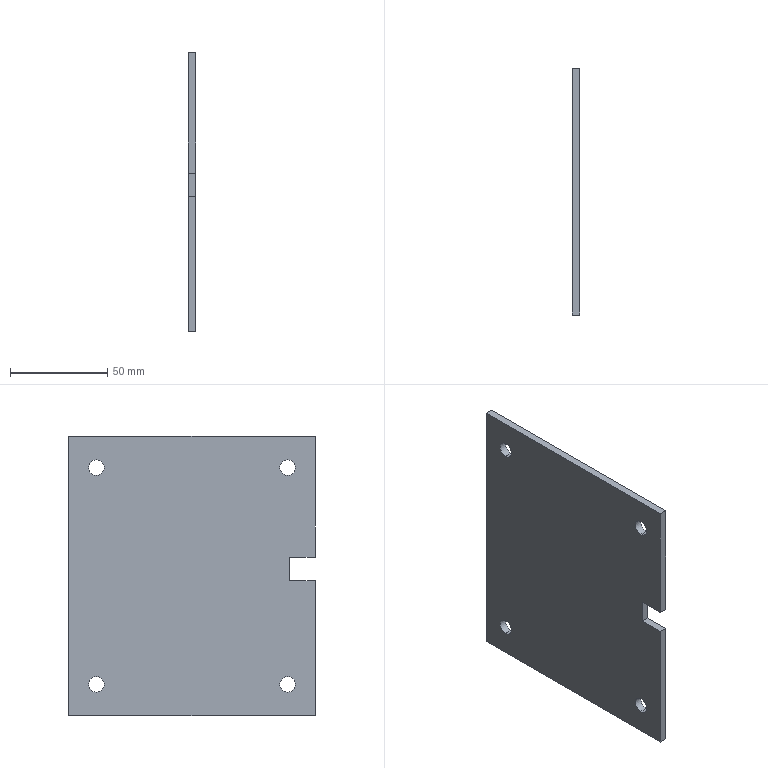Component | SolidWorks | Part1^Assembly2-1 | 1 solid | 18 faces | box 4 x 127 x 144 mm | volume 71714 mm3 | plane 10 | cylinder 8 | commonest cylinder face diameters 8 x8
STEP:
#1=COLOUR_RGB('',0.7922,0.8196,0.9333);
#2=FILL_AREA_STYLE_COLOUR('',#1);
#3=FILL_AREA_STYLE('',(#2));
#4=SURFACE_STYLE_FILL_AREA(#3);
#5=SURFACE_SIDE_STYLE('',(#4));
#6=SURFACE_STYLE_USAGE(.BOTH.,#5);
#7=PRESENTATION_STYLE_ASSIGNMENT((#6));
#8=CARTESIAN_POINT('',(5.984,11.308,-14.024));
#9=VERTEX_POINT('',#8);
#10=CARTESIAN_POINT('',(5.984,11.308,-14.339));
#11=VERTEX_POINT('',#10);
#12=CARTESIAN_POINT('',(5.984,11.308,-14.182));
#13=DIRECTION('',(1.,0.,0.));
#14=DIRECTION('',(0.,0.,-1.));
#15=AXIS2_PLACEMENT_3D('',#12,#13,#14);
#16=CIRCLE('',#15,0.1575);
#17=EDGE_CURVE('',#9,#11,#16,.T.);
#18=ORIENTED_EDGE('',*,*,#17,.T.);
#19=CARTESIAN_POINT('',(5.827,11.308,-14.339));
#20=VERTEX_POINT('',#19);
#21=CARTESIAN_POINT('',(5.984,11.308,-14.339));
#22=DIRECTION('',(-1.,0.,0.));
#23=VECTOR('',#22,39.37);
#24=LINE('',#21,#23);
#25=EDGE_CURVE('',#11,#20,#24,.T.);
#26=ORIENTED_EDGE('',*,*,#25,.T.);
#27=CARTESIAN_POINT('',(5.827,11.308,-14.024));
#28=VERTEX_POINT('',#27);
#29=CARTESIAN_POINT('',(5.827,11.308,-14.182));
#30=DIRECTION('',(1.,0.,0.));
#31=DIRECTION('',(0.,0.,-1.));
#32=AXIS2_PLACEMENT_3D('',#29,#30,#31);
#33=CIRCLE('',#32,0.1575);
#34=EDGE_CURVE('',#28,#20,#33,.T.);
#35=ORIENTED_EDGE('',*,*,#34,.F.);
#36=CARTESIAN_POINT('',(5.984,11.308,-14.024));
#37=DIRECTION('',(-1.,0.,0.));
#38=VECTOR('',#37,39.37);
#39=LINE('',#36,#38);
#40=EDGE_CURVE('',#9,#28,#39,.T.);
#41=ORIENTED_EDGE('',*,*,#40,.F.);
#42=EDGE_LOOP('',(#18,#26,#35,#41));
#43=FACE_OUTER_BOUND('',#42,.T.);
#44=CARTESIAN_POINT('',(5.984,11.308,-14.182));
#45=DIRECTION('',(-1.,0.,0.));
#46=DIRECTION('',(0.,0.,1.));
#47=AXIS2_PLACEMENT_3D('',#44,#45,#46);
#48=CYLINDRICAL_SURFACE('',#47,0.1575);
#49=ADVANCED_FACE('',(#43),#48,.F.);
#50=CARTESIAN_POINT('',(5.984,11.308,-18.424));
#51=VERTEX_POINT('',#50);
#52=CARTESIAN_POINT('',(5.984,11.308,-18.739));
#53=VERTEX_POINT('',#52);
#54=CARTESIAN_POINT('',(5.984,11.308,-18.581));
#55=DIRECTION('',(1.,0.,0.));
#56=DIRECTION('',(0.,0.,-1.));
#57=AXIS2_PLACEMENT_3D('',#54,#55,#56);
#58=CIRCLE('',#57,0.1575);
#59=EDGE_CURVE('',#51,#53,#58,.T.);
#60=ORIENTED_EDGE('',*,*,#59,.T.);
#61=CARTESIAN_POINT('',(5.827,11.308,-18.739));
#62=VERTEX_POINT('',#61);
#63=CARTESIAN_POINT('',(5.984,11.308,-18.739));
#64=DIRECTION('',(-1.,0.,0.));
#65=VECTOR('',#64,39.37);
#66=LINE('',#63,#65);
#67=EDGE_CURVE('',#53,#62,#66,.T.);
#68=ORIENTED_EDGE('',*,*,#67,.T.);
#69=CARTESIAN_POINT('',(5.827,11.308,-18.424));
#70=VERTEX_POINT('',#69);
#71=CARTESIAN_POINT('',(5.827,11.308,-18.581));
#72=DIRECTION('',(1.,0.,0.));
#73=DIRECTION('',(0.,0.,-1.));
#74=AXIS2_PLACEMENT_3D('',#71,#72,#73);
#75=CIRCLE('',#74,0.1575);
#76=EDGE_CURVE('',#70,#62,#75,.T.);
#77=ORIENTED_EDGE('',*,*,#76,.F.);
#78=CARTESIAN_POINT('',(5.984,11.308,-18.424));
#79=DIRECTION('',(-1.,0.,0.));
#80=VECTOR('',#79,39.37);
#81=LINE('',#78,#80);
#82=EDGE_CURVE('',#51,#70,#81,.T.);
#83=ORIENTED_EDGE('',*,*,#82,.F.);
#84=EDGE_LOOP('',(#60,#68,#77,#83));
#85=FACE_OUTER_BOUND('',#84,.T.);
#86=CARTESIAN_POINT('',(5.984,11.308,-18.581));
#87=DIRECTION('',(-1.,0.,0.));
#88=DIRECTION('',(0.,0.,1.));
#89=AXIS2_PLACEMENT_3D('',#86,#87,#88);
#90=CYLINDRICAL_SURFACE('',#89,0.1575);
#91=ADVANCED_FACE('',(#85),#90,.F.);
#92=CARTESIAN_POINT('',(5.984,15.188,-18.424));
#93=VERTEX_POINT('',#92);
#94=CARTESIAN_POINT('',(5.984,15.188,-18.739));
#95=VERTEX_POINT('',#94);
#96=CARTESIAN_POINT('',(5.984,15.188,-18.581));
#97=DIRECTION('',(1.,0.,0.));
#98=DIRECTION('',(0.,0.,-1.));
#99=AXIS2_PLACEMENT_3D('',#96,#97,#98);
#100=CIRCLE('',#99,0.1575);
#101=EDGE_CURVE('',#93,#95,#100,.T.);
#102=ORIENTED_EDGE('',*,*,#101,.T.);
#103=CARTESIAN_POINT('',(5.827,15.188,-18.739));
#104=VERTEX_POINT('',#103);
#105=CARTESIAN_POINT('',(5.984,15.188,-18.739));
#106=DIRECTION('',(-1.,0.,0.));
#107=VECTOR('',#106,39.37);
#108=LINE('',#105,#107);
#109=EDGE_CURVE('',#95,#104,#108,.T.);
#110=ORIENTED_EDGE('',*,*,#109,.T.);
#111=CARTESIAN_POINT('',(5.827,15.188,-18.424));
#112=VERTEX_POINT('',#111);
#113=CARTESIAN_POINT('',(5.827,15.188,-18.581));
#114=DIRECTION('',(1.,0.,0.));
#115=DIRECTION('',(0.,0.,-1.));
#116=AXIS2_PLACEMENT_3D('',#113,#114,#115);
#117=CIRCLE('',#116,0.1575);
#118=EDGE_CURVE('',#112,#104,#117,.T.);
#119=ORIENTED_EDGE('',*,*,#118,.F.);
#120=CARTESIAN_POINT('',(5.984,15.188,-18.424));
#121=DIRECTION('',(-1.,0.,0.));
#122=VECTOR('',#121,39.37);
#123=LINE('',#120,#122);
#124=EDGE_CURVE('',#93,#112,#123,.T.);
#125=ORIENTED_EDGE('',*,*,#124,.F.);
#126=EDGE_LOOP('',(#102,#110,#119,#125));
#127=FACE_OUTER_BOUND('',#126,.T.);
#128=CARTESIAN_POINT('',(5.984,15.188,-18.581));
#129=DIRECTION('',(-1.,0.,0.));
#130=DIRECTION('',(0.,0.,1.));
#131=AXIS2_PLACEMENT_3D('',#128,#129,#130);
#132=CYLINDRICAL_SURFACE('',#131,0.1575);
#133=ADVANCED_FACE('',(#127),#132,.F.);
#134=CARTESIAN_POINT('',(5.984,15.188,-14.024));
#135=VERTEX_POINT('',#134);
#136=CARTESIAN_POINT('',(5.984,15.188,-14.339));
#137=VERTEX_POINT('',#136);
#138=CARTESIAN_POINT('',(5.984,15.188,-14.182));
#139=DIRECTION('',(1.,0.,0.));
#140=DIRECTION('',(0.,0.,-1.));
#141=AXIS2_PLACEMENT_3D('',#138,#139,#140);
#142=CIRCLE('',#141,0.1575);
#143=EDGE_CURVE('',#135,#137,#142,.T.);
#144=ORIENTED_EDGE('',*,*,#143,.T.);
#145=CARTESIAN_POINT('',(5.827,15.188,-14.339));
#146=VERTEX_POINT('',#145);
#147=CARTESIAN_POINT('',(5.984,15.188,-14.339));
#148=DIRECTION('',(-1.,0.,0.));
#149=VECTOR('',#148,39.37);
#150=LINE('',#147,#149);
#151=EDGE_CURVE('',#137,#146,#150,.T.);
#152=ORIENTED_EDGE('',*,*,#151,.T.);
#153=CARTESIAN_POINT('',(5.827,15.188,-14.024));
#154=VERTEX_POINT('',#153);
#155=CARTESIAN_POINT('',(5.827,15.188,-14.182));
#156=DIRECTION('',(1.,0.,0.));
#157=DIRECTION('',(0.,0.,-1.));
#158=AXIS2_PLACEMENT_3D('',#155,#156,#157);
#159=CIRCLE('',#158,0.1575);
#160=EDGE_CURVE('',#154,#146,#159,.T.);
#161=ORIENTED_EDGE('',*,*,#160,.F.);
#162=CARTESIAN_POINT('',(5.984,15.188,-14.024));
#163=DIRECTION('',(-1.,0.,0.));
#164=VECTOR('',#163,39.37);
#165=LINE('',#162,#164);
#166=EDGE_CURVE('',#135,#154,#165,.T.);
#167=ORIENTED_EDGE('',*,*,#166,.F.);
#168=EDGE_LOOP('',(#144,#152,#161,#167));
#169=FACE_OUTER_BOUND('',#168,.T.);
#170=CARTESIAN_POINT('',(5.984,15.188,-14.182));
#171=DIRECTION('',(-1.,0.,0.));
#172=DIRECTION('',(0.,0.,1.));
#173=AXIS2_PLACEMENT_3D('',#170,#171,#172);
#174=CYLINDRICAL_SURFACE('',#173,0.1575);
#175=ADVANCED_FACE('',(#169),#174,.F.);
#176=ORIENTED_EDGE('',*,*,#17,.F.);
#177=CARTESIAN_POINT('',(5.984,11.308,-14.182));
#178=DIRECTION('',(1.,0.,0.));
#179=DIRECTION('',(0.,0.,-1.));
#180=AXIS2_PLACEMENT_3D('',#177,#178,#179);
#181=CIRCLE('',#180,0.1575);
#182=EDGE_CURVE('',#11,#9,#181,.T.);
#183=ORIENTED_EDGE('',*,*,#182,.F.);
#184=EDGE_LOOP('',(#176,#183));
#185=FACE_BOUND('',#184,.T.);
#186=ORIENTED_EDGE('',*,*,#59,.F.);
#187=CARTESIAN_POINT('',(5.984,11.308,-18.581));
#188=DIRECTION('',(1.,0.,0.));
#189=DIRECTION('',(0.,0.,-1.));
#190=AXIS2_PLACEMENT_3D('',#187,#188,#189);
#191=CIRCLE('',#190,0.1575);
#192=EDGE_CURVE('',#53,#51,#191,.T.);
#193=ORIENTED_EDGE('',*,*,#192,.F.);
#194=EDGE_LOOP('',(#186,#193));
#195=FACE_BOUND('',#194,.T.);
#196=ORIENTED_EDGE('',*,*,#101,.F.);
#197=CARTESIAN_POINT('',(5.984,15.188,-18.581));
#198=DIRECTION('',(1.,0.,0.));
#199=DIRECTION('',(0.,0.,-1.));
#200=AXIS2_PLACEMENT_3D('',#197,#198,#199);
#201=CIRCLE('',#200,0.1575);
#202=EDGE_CURVE('',#95,#93,#201,.T.);
#203=ORIENTED_EDGE('',*,*,#202,.F.);
#204=EDGE_LOOP('',(#196,#203));
#205=FACE_BOUND('',#204,.T.);
#206=ORIENTED_EDGE('',*,*,#143,.F.);
#207=CARTESIAN_POINT('',(5.984,15.188,-14.182));
#208=DIRECTION('',(1.,0.,0.));
#209=DIRECTION('',(0.,0.,-1.));
#210=AXIS2_PLACEMENT_3D('',#207,#208,#209);
#211=CIRCLE('',#210,0.1575);
#212=EDGE_CURVE('',#137,#135,#211,.T.);
#213=ORIENTED_EDGE('',*,*,#212,.F.);
#214=EDGE_LOOP('',(#206,#213));
#215=FACE_BOUND('',#214,.T.);
#216=CARTESIAN_POINT('',(5.984,11.269,-16.001));
#217=VERTEX_POINT('',#216);
#218=CARTESIAN_POINT('',(5.984,10.748,-16.001));
#219=VERTEX_POINT('',#218);
#220=CARTESIAN_POINT('',(5.984,10.433,-16.001));
#221=DIRECTION('',(0.,-1.,0.));
#222=VECTOR('',#221,39.37);
#223=LINE('',#220,#222);
#224=EDGE_CURVE('',#217,#219,#223,.T.);
#225=ORIENTED_EDGE('',*,*,#224,.F.);
#226=CARTESIAN_POINT('',(5.984,11.269,-16.474));
#227=VERTEX_POINT('',#226);
#228=CARTESIAN_POINT('',(5.984,11.269,-16.001));
#229=DIRECTION('',(0.,0.,1.));
#230=VECTOR('',#229,39.37);
#231=LINE('',#228,#230);
#232=EDGE_CURVE('',#227,#217,#231,.T.);
#233=ORIENTED_EDGE('',*,*,#232,.F.);
#234=CARTESIAN_POINT('',(5.984,10.748,-16.474));
#235=VERTEX_POINT('',#234);
#236=CARTESIAN_POINT('',(5.984,10.433,-16.474));
#237=DIRECTION('',(0.,1.,0.));
#238=VECTOR('',#237,39.37);
#239=LINE('',#236,#238);
#240=EDGE_CURVE('',#235,#227,#239,.T.);
#241=ORIENTED_EDGE('',*,*,#240,.F.);
#242=CARTESIAN_POINT('',(5.984,10.748,-19.216));
#243=VERTEX_POINT('',#242);
#244=CARTESIAN_POINT('',(5.984,10.748,-19.216));
#245=DIRECTION('',(0.,0.,-1.));
#246=VECTOR('',#245,39.37);
#247=LINE('',#244,#246);
#248=EDGE_CURVE('',#235,#243,#247,.T.);
#249=ORIENTED_EDGE('',*,*,#248,.T.);
#250=CARTESIAN_POINT('',(5.984,15.748,-19.216));
#251=VERTEX_POINT('',#250);
#252=CARTESIAN_POINT('',(5.984,15.748,-19.216));
#253=DIRECTION('',(0.,1.,0.));
#254=VECTOR('',#253,39.37);
#255=LINE('',#252,#254);
#256=EDGE_CURVE('',#243,#251,#255,.T.);
#257=ORIENTED_EDGE('',*,*,#256,.T.);
#258=CARTESIAN_POINT('',(5.984,15.748,-13.547));
#259=VERTEX_POINT('',#258);
#260=CARTESIAN_POINT('',(5.984,15.748,-19.216));
#261=DIRECTION('',(0.,0.,1.));
#262=VECTOR('',#261,39.37);
#263=LINE('',#260,#262);
#264=EDGE_CURVE('',#251,#259,#263,.T.);
#265=ORIENTED_EDGE('',*,*,#264,.T.);
#266=CARTESIAN_POINT('',(5.984,10.748,-13.547));
#267=VERTEX_POINT('',#266);
#268=CARTESIAN_POINT('',(5.984,15.748,-13.547));
#269=DIRECTION('',(0.,-1.,0.));
#270=VECTOR('',#269,39.37);
#271=LINE('',#268,#270);
#272=EDGE_CURVE('',#259,#267,#271,.T.);
#273=ORIENTED_EDGE('',*,*,#272,.T.);
#274=CARTESIAN_POINT('',(5.984,10.748,-19.216));
#275=DIRECTION('',(0.,0.,-1.));
#276=VECTOR('',#275,39.37);
#277=LINE('',#274,#276);
#278=EDGE_CURVE('',#267,#219,#277,.T.);
#279=ORIENTED_EDGE('',*,*,#278,.T.);
#280=EDGE_LOOP('',(#225,#233,#241,#249,#257,#265,#273,#279));
#281=FACE_OUTER_BOUND('',#280,.T.);
#282=CARTESIAN_POINT('',(5.984,2.585,-8.629));
#283=DIRECTION('',(-1.,0.,0.));
#284=DIRECTION('',(0.,0.,1.));
#285=AXIS2_PLACEMENT_3D('',#282,#283,#284);
#286=PLANE('',#285);
#287=ADVANCED_FACE('',(#185,#195,#205,#215,#281),#286,.F.);
#288=ORIENTED_EDGE('',*,*,#76,.T.);
#289=CARTESIAN_POINT('',(5.827,11.308,-18.581));
#290=DIRECTION('',(1.,0.,0.));
#291=DIRECTION('',(0.,0.,-1.));
#292=AXIS2_PLACEMENT_3D('',#289,#290,#291);
#293=CIRCLE('',#292,0.1575);
#294=EDGE_CURVE('',#62,#70,#293,.T.);
#295=ORIENTED_EDGE('',*,*,#294,.T.);
#296=EDGE_LOOP('',(#288,#295));
#297=FACE_BOUND('',#296,.T.);
#298=ORIENTED_EDGE('',*,*,#160,.T.);
#299=CARTESIAN_POINT('',(5.827,15.188,-14.182));
#300=DIRECTION('',(1.,0.,0.));
#301=DIRECTION('',(0.,0.,-1.));
#302=AXIS2_PLACEMENT_3D('',#299,#300,#301);
#303=CIRCLE('',#302,0.1575);
#304=EDGE_CURVE('',#146,#154,#303,.T.);
#305=ORIENTED_EDGE('',*,*,#304,.T.);
#306=EDGE_LOOP('',(#298,#305));
#307=FACE_BOUND('',#306,.T.);
#308=ORIENTED_EDGE('',*,*,#118,.T.);
#309=CARTESIAN_POINT('',(5.827,15.188,-18.581));
#310=DIRECTION('',(1.,0.,0.));
#311=DIRECTION('',(0.,0.,-1.));
#312=AXIS2_PLACEMENT_3D('',#309,#310,#311);
#313=CIRCLE('',#312,0.1575);
#314=EDGE_CURVE('',#104,#112,#313,.T.);
#315=ORIENTED_EDGE('',*,*,#314,.T.);
#316=EDGE_LOOP('',(#308,#315));
#317=FACE_BOUND('',#316,.T.);
#318=ORIENTED_EDGE('',*,*,#34,.T.);
#319=CARTESIAN_POINT('',(5.827,11.308,-14.182));
#320=DIRECTION('',(1.,0.,0.));
#321=DIRECTION('',(0.,0.,-1.));
#322=AXIS2_PLACEMENT_3D('',#319,#320,#321);
#323=CIRCLE('',#322,0.1575);
#324=EDGE_CURVE('',#20,#28,#323,.T.);
#325=ORIENTED_EDGE('',*,*,#324,.T.);
#326=EDGE_LOOP('',(#318,#325));
#327=FACE_BOUND('',#326,.T.);
#328=CARTESIAN_POINT('',(5.827,11.269,-16.474));
#329=VERTEX_POINT('',#328);
#330=CARTESIAN_POINT('',(5.827,11.269,-16.001));
#331=VERTEX_POINT('',#330);
#332=CARTESIAN_POINT('',(5.827,11.269,-16.001));
#333=DIRECTION('',(0.,0.,1.));
#334=VECTOR('',#333,39.37);
#335=LINE('',#332,#334);
#336=EDGE_CURVE('',#329,#331,#335,.T.);
#337=ORIENTED_EDGE('',*,*,#336,.T.);
#338=CARTESIAN_POINT('',(5.827,10.748,-16.001));
#339=VERTEX_POINT('',#338);
#340=CARTESIAN_POINT('',(5.827,10.433,-16.001));
#341=DIRECTION('',(0.,-1.,0.));
#342=VECTOR('',#341,39.37);
#343=LINE('',#340,#342);
#344=EDGE_CURVE('',#331,#339,#343,.T.);
#345=ORIENTED_EDGE('',*,*,#344,.T.);
#346=CARTESIAN_POINT('',(5.827,10.748,-13.547));
#347=VERTEX_POINT('',#346);
#348=CARTESIAN_POINT('',(5.827,10.748,-19.216));
#349=DIRECTION('',(0.,0.,-1.));
#350=VECTOR('',#349,39.37);
#351=LINE('',#348,#350);
#352=EDGE_CURVE('',#347,#339,#351,.T.);
#353=ORIENTED_EDGE('',*,*,#352,.F.);
#354=CARTESIAN_POINT('',(5.827,15.748,-13.547));
#355=VERTEX_POINT('',#354);
#356=CARTESIAN_POINT('',(5.827,15.748,-13.547));
#357=DIRECTION('',(0.,-1.,0.));
#358=VECTOR('',#357,39.37);
#359=LINE('',#356,#358);
#360=EDGE_CURVE('',#355,#347,#359,.T.);
#361=ORIENTED_EDGE('',*,*,#360,.F.);
#362=CARTESIAN_POINT('',(5.827,15.748,-19.216));
#363=VERTEX_POINT('',#362);
#364=CARTESIAN_POINT('',(5.827,15.748,-19.216));
#365=DIRECTION('',(0.,0.,1.));
#366=VECTOR('',#365,39.37);
#367=LINE('',#364,#366);
#368=EDGE_CURVE('',#363,#355,#367,.T.);
#369=ORIENTED_EDGE('',*,*,#368,.F.);
#370=CARTESIAN_POINT('',(5.827,10.748,-19.216));
#371=VERTEX_POINT('',#370);
#372=CARTESIAN_POINT('',(5.827,15.748,-19.216));
#373=DIRECTION('',(0.,1.,0.));
#374=VECTOR('',#373,39.37);
#375=LINE('',#372,#374);
#376=EDGE_CURVE('',#371,#363,#375,.T.);
#377=ORIENTED_EDGE('',*,*,#376,.F.);
#378=CARTESIAN_POINT('',(5.827,10.748,-16.474));
#379=VERTEX_POINT('',#378);
#380=CARTESIAN_POINT('',(5.827,10.748,-19.216));
#381=DIRECTION('',(0.,0.,-1.));
#382=VECTOR('',#381,39.37);
#383=LINE('',#380,#382);
#384=EDGE_CURVE('',#379,#371,#383,.T.);
#385=ORIENTED_EDGE('',*,*,#384,.F.);
#386=CARTESIAN_POINT('',(5.827,10.433,-16.474));
#387=DIRECTION('',(0.,1.,0.));
#388=VECTOR('',#387,39.37);
#389=LINE('',#386,#388);
#390=EDGE_CURVE('',#379,#329,#389,.T.);
#391=ORIENTED_EDGE('',*,*,#390,.T.);
#392=EDGE_LOOP('',(#337,#345,#353,#361,#369,#377,#385,#391));
#393=FACE_OUTER_BOUND('',#392,.T.);
#394=CARTESIAN_POINT('',(5.827,2.585,-8.629));
#395=DIRECTION('',(-1.,0.,0.));
#396=DIRECTION('',(0.,0.,1.));
#397=AXIS2_PLACEMENT_3D('',#394,#395,#396);
#398=PLANE('',#397);
#399=ADVANCED_FACE('',(#297,#307,#317,#327,#393),#398,.T.);
#400=ORIENTED_EDGE('',*,*,#352,.T.);
#401=CARTESIAN_POINT('',(5.984,10.748,-16.001));
#402=DIRECTION('',(1.,0.,0.));
#403=VECTOR('',#402,39.37);
#404=LINE('',#401,#403);
#405=EDGE_CURVE('',#339,#219,#404,.T.);
#406=ORIENTED_EDGE('',*,*,#405,.T.);
#407=ORIENTED_EDGE('',*,*,#278,.F.);
#408=CARTESIAN_POINT('',(5.984,10.748,-13.547));
#409=DIRECTION('',(-1.,0.,0.));
#410=VECTOR('',#409,39.37);
#411=LINE('',#408,#410);
#412=EDGE_CURVE('',#267,#347,#411,.T.);
#413=ORIENTED_EDGE('',*,*,#412,.T.);
#414=EDGE_LOOP('',(#400,#406,#407,#413));
#415=FACE_OUTER_BOUND('',#414,.T.);
#416=CARTESIAN_POINT('',(5.984,10.748,-19.216));
#417=DIRECTION('',(0.,1.,0.));
#418=DIRECTION('',(1.,0.,0.));
#419=AXIS2_PLACEMENT_3D('',#416,#417,#418);
#420=PLANE('',#419);
#421=ADVANCED_FACE('',(#415),#420,.F.);
#422=ORIENTED_EDGE('',*,*,#360,.T.);
#423=ORIENTED_EDGE('',*,*,#412,.F.);
#424=ORIENTED_EDGE('',*,*,#272,.F.);
#425=CARTESIAN_POINT('',(5.984,15.748,-13.547));
#426=DIRECTION('',(-1.,0.,0.));
#427=VECTOR('',#426,39.37);
#428=LINE('',#425,#427);
#429=EDGE_CURVE('',#259,#355,#428,.T.);
#430=ORIENTED_EDGE('',*,*,#429,.T.);
#431=EDGE_LOOP('',(#422,#423,#424,#430));
#432=FACE_OUTER_BOUND('',#431,.T.);
#433=CARTESIAN_POINT('',(5.984,15.748,-13.547));
#434=DIRECTION('',(0.,0.,-1.));
#435=DIRECTION('',(-1.,0.,0.));
#436=AXIS2_PLACEMENT_3D('',#433,#434,#435);
#437=PLANE('',#436);
#438=ADVANCED_FACE('',(#432),#437,.F.);
#439=ORIENTED_EDGE('',*,*,#248,.F.);
#440=CARTESIAN_POINT('',(5.984,10.748,-16.474));
#441=DIRECTION('',(-1.,0.,0.));
#442=VECTOR('',#441,39.37);
#443=LINE('',#440,#442);
#444=EDGE_CURVE('',#235,#379,#443,.T.);
#445=ORIENTED_EDGE('',*,*,#444,.T.);
#446=ORIENTED_EDGE('',*,*,#384,.T.);
#447=CARTESIAN_POINT('',(5.984,10.748,-19.216));
#448=DIRECTION('',(-1.,0.,0.));
#449=VECTOR('',#448,39.37);
#450=LINE('',#447,#449);
#451=EDGE_CURVE('',#243,#371,#450,.T.);
#452=ORIENTED_EDGE('',*,*,#451,.F.);
#453=EDGE_LOOP('',(#439,#445,#446,#452));
#454=FACE_OUTER_BOUND('',#453,.T.);
#455=CARTESIAN_POINT('',(5.984,10.748,-19.216));
#456=DIRECTION('',(0.,1.,0.));
#457=DIRECTION('',(1.,0.,0.));
#458=AXIS2_PLACEMENT_3D('',#455,#456,#457);
#459=PLANE('',#458);
#460=ADVANCED_FACE('',(#454),#459,.F.);
#461=ORIENTED_EDGE('',*,*,#376,.T.);
#462=CARTESIAN_POINT('',(5.984,15.748,-19.216));
#463=DIRECTION('',(-1.,0.,0.));
#464=VECTOR('',#463,39.37);
#465=LINE('',#462,#464);
#466=EDGE_CURVE('',#251,#363,#465,.T.);
#467=ORIENTED_EDGE('',*,*,#466,.F.);
#468=ORIENTED_EDGE('',*,*,#256,.F.);
#469=ORIENTED_EDGE('',*,*,#451,.T.);
#470=EDGE_LOOP('',(#461,#467,#468,#469));
#471=FACE_OUTER_BOUND('',#470,.T.);
#472=CARTESIAN_POINT('',(5.984,15.748,-19.216));
#473=DIRECTION('',(0.,0.,1.));
#474=DIRECTION('',(1.,0.,0.));
#475=AXIS2_PLACEMENT_3D('',#472,#473,#474);
#476=PLANE('',#475);
#477=ADVANCED_FACE('',(#471),#476,.F.);
#478=ORIENTED_EDGE('',*,*,#368,.T.);
#479=ORIENTED_EDGE('',*,*,#429,.F.);
#480=ORIENTED_EDGE('',*,*,#264,.F.);
#481=ORIENTED_EDGE('',*,*,#466,.T.);
#482=EDGE_LOOP('',(#478,#479,#480,#481));
#483=FACE_OUTER_BOUND('',#482,.T.);
#484=CARTESIAN_POINT('',(5.984,15.748,-19.216));
#485=DIRECTION('',(0.,-1.,0.));
#486=DIRECTION('',(-1.,0.,0.));
#487=AXIS2_PLACEMENT_3D('',#484,#485,#486);
#488=PLANE('',#487);
#489=ADVANCED_FACE('',(#483),#488,.F.);
#490=ORIENTED_EDGE('',*,*,#151,.F.);
#491=ORIENTED_EDGE('',*,*,#212,.T.);
#492=ORIENTED_EDGE('',*,*,#166,.T.);
#493=ORIENTED_EDGE('',*,*,#304,.F.);
#494=EDGE_LOOP('',(#490,#491,#492,#493));
#495=FACE_OUTER_BOUND('',#494,.T.);
#496=CARTESIAN_POINT('',(5.984,15.188,-14.182));
#497=DIRECTION('',(-1.,0.,0.));
#498=DIRECTION('',(0.,0.,1.));
#499=AXIS2_PLACEMENT_3D('',#496,#497,#498);
#500=CYLINDRICAL_SURFACE('',#499,0.1575);
#501=ADVANCED_FACE('',(#495),#500,.F.);
#502=ORIENTED_EDGE('',*,*,#109,.F.);
#503=ORIENTED_EDGE('',*,*,#202,.T.);
#504=ORIENTED_EDGE('',*,*,#124,.T.);
#505=ORIENTED_EDGE('',*,*,#314,.F.);
#506=EDGE_LOOP('',(#502,#503,#504,#505));
#507=FACE_OUTER_BOUND('',#506,.T.);
#508=CARTESIAN_POINT('',(5.984,15.188,-18.581));
#509=DIRECTION('',(-1.,0.,0.));
#510=DIRECTION('',(0.,0.,1.));
#511=AXIS2_PLACEMENT_3D('',#508,#509,#510);
#512=CYLINDRICAL_SURFACE('',#511,0.1575);
#513=ADVANCED_FACE('',(#507),#512,.F.);
#514=ORIENTED_EDGE('',*,*,#67,.F.);
#515=ORIENTED_EDGE('',*,*,#192,.T.);
#516=ORIENTED_EDGE('',*,*,#82,.T.);
#517=ORIENTED_EDGE('',*,*,#294,.F.);
#518=EDGE_LOOP('',(#514,#515,#516,#517));
#519=FACE_OUTER_BOUND('',#518,.T.);
#520=CARTESIAN_POINT('',(5.984,11.308,-18.581));
#521=DIRECTION('',(-1.,0.,0.));
#522=DIRECTION('',(0.,0.,1.));
#523=AXIS2_PLACEMENT_3D('',#520,#521,#522);
#524=CYLINDRICAL_SURFACE('',#523,0.1575);
#525=ADVANCED_FACE('',(#519),#524,.F.);
#526=ORIENTED_EDGE('',*,*,#25,.F.);
#527=ORIENTED_EDGE('',*,*,#182,.T.);
#528=ORIENTED_EDGE('',*,*,#40,.T.);
#529=ORIENTED_EDGE('',*,*,#324,.F.);
#530=EDGE_LOOP('',(#526,#527,#528,#529));
#531=FACE_OUTER_BOUND('',#530,.T.);
#532=CARTESIAN_POINT('',(5.984,11.308,-14.182));
#533=DIRECTION('',(-1.,0.,0.));
#534=DIRECTION('',(0.,0.,1.));
#535=AXIS2_PLACEMENT_3D('',#532,#533,#534);
#536=CYLINDRICAL_SURFACE('',#535,0.1575);
#537=ADVANCED_FACE('',(#531),#536,.F.);
#538=ORIENTED_EDGE('',*,*,#344,.F.);
#539=CARTESIAN_POINT('',(5.827,11.269,-16.001));
#540=DIRECTION('',(1.,0.,0.));
#541=VECTOR('',#540,39.37);
#542=LINE('',#539,#541);
#543=EDGE_CURVE('',#331,#217,#542,.T.);
#544=ORIENTED_EDGE('',*,*,#543,.T.);
#545=ORIENTED_EDGE('',*,*,#224,.T.);
#546=ORIENTED_EDGE('',*,*,#405,.F.);
#547=EDGE_LOOP('',(#538,#544,#545,#546));
#548=FACE_OUTER_BOUND('',#547,.T.);
#549=CARTESIAN_POINT('',(5.827,10.433,-16.001));
#550=DIRECTION('',(0.,0.,1.));
#551=DIRECTION('',(1.,0.,0.));
#552=AXIS2_PLACEMENT_3D('',#549,#550,#551);
#553=PLANE('',#552);
#554=ADVANCED_FACE('',(#548),#553,.F.);
#555=ORIENTED_EDGE('',*,*,#240,.T.);
#556=CARTESIAN_POINT('',(5.827,11.269,-16.474));
#557=DIRECTION('',(1.,0.,0.));
#558=VECTOR('',#557,39.37);
#559=LINE('',#556,#558);
#560=EDGE_CURVE('',#329,#227,#559,.T.);
#561=ORIENTED_EDGE('',*,*,#560,.F.);
#562=ORIENTED_EDGE('',*,*,#390,.F.);
#563=ORIENTED_EDGE('',*,*,#444,.F.);
#564=EDGE_LOOP('',(#555,#561,#562,#563));
#565=FACE_OUTER_BOUND('',#564,.T.);
#566=CARTESIAN_POINT('',(5.827,10.433,-16.474));
#567=DIRECTION('',(0.,0.,-1.));
#568=DIRECTION('',(-1.,0.,0.));
#569=AXIS2_PLACEMENT_3D('',#566,#567,#568);
#570=PLANE('',#569);
#571=ADVANCED_FACE('',(#565),#570,.F.);
#572=ORIENTED_EDGE('',*,*,#543,.F.);
#573=ORIENTED_EDGE('',*,*,#336,.F.);
#574=ORIENTED_EDGE('',*,*,#560,.T.);
#575=ORIENTED_EDGE('',*,*,#232,.T.);
#576=EDGE_LOOP('',(#572,#573,#574,#575));
#577=FACE_OUTER_BOUND('',#576,.T.);
#578=CARTESIAN_POINT('',(5.827,11.269,-16.001));
#579=DIRECTION('',(0.,1.,0.));
#580=DIRECTION('',(1.,0.,0.));
#581=AXIS2_PLACEMENT_3D('',#578,#579,#580);
#582=PLANE('',#581);
#583=ADVANCED_FACE('',(#577),#582,.F.);
#584=CLOSED_SHELL('',(#49,#91,#133,#175,#287,#399,#421,#438,#460,#477,#489,#501,#513,#525,#537,#554,#571,#583));
#585=MANIFOLD_SOLID_BREP('',#584);
#586=STYLED_ITEM('',(#7),#585);
#587=PRESENTATION_LAYER_ASSIGNMENT('','',(#586));
#588=CARTESIAN_POINT('',(0.,0.,0.));
#589=DIRECTION('',(0.,0.,1.));
#590=DIRECTION('',(1.,0.,0.));
#591=AXIS2_PLACEMENT_3D('',#588,#589,#590);
#592=(LENGTH_UNIT()NAMED_UNIT(*)SI_UNIT($,.METRE.));
#593=LENGTH_MEASURE_WITH_UNIT(LENGTH_MEASURE(0.0254),#592);
#594=DIMENSIONAL_EXPONENTS(1.,0.,0.,0.,0.,0.,0.);
#595=(CONVERSION_BASED_UNIT('',#593)LENGTH_UNIT()NAMED_UNIT(#594));
#596=UNCERTAINTY_MEASURE_WITH_UNIT(LENGTH_MEASURE(0.00001),#595,'','');
#597=(NAMED_UNIT(*)PLANE_ANGLE_UNIT()SI_UNIT($,.RADIAN.));
#598=(NAMED_UNIT(*)SI_UNIT($,.STERADIAN.)SOLID_ANGLE_UNIT());
#599=(GEOMETRIC_REPRESENTATION_CONTEXT(3)GLOBAL_UNCERTAINTY_ASSIGNED_CONTEXT((#596))GLOBAL_UNIT_ASSIGNED_CONTEXT((#595,#597,#598))REPRESENTATION_CONTEXT('',''));
#600=ADVANCED_BREP_SHAPE_REPRESENTATION('',(#585,#591),#599);
#601=(LENGTH_UNIT()NAMED_UNIT(*)SI_UNIT($,.METRE.));
#602=LENGTH_MEASURE_WITH_UNIT(LENGTH_MEASURE(0.0254),#601);
#603=DIMENSIONAL_EXPONENTS(1.,0.,0.,0.,0.,0.,0.);
#604=(CONVERSION_BASED_UNIT('',#602)LENGTH_UNIT()NAMED_UNIT(#603));
#605=UNCERTAINTY_MEASURE_WITH_UNIT(LENGTH_MEASURE(0.00001),#604,'','');
#606=(NAMED_UNIT(*)PLANE_ANGLE_UNIT()SI_UNIT($,.RADIAN.));
#607=(NAMED_UNIT(*)SI_UNIT($,.STERADIAN.)SOLID_ANGLE_UNIT());
#608=(GEOMETRIC_REPRESENTATION_CONTEXT(3)GLOBAL_UNCERTAINTY_ASSIGNED_CONTEXT((#605))GLOBAL_UNIT_ASSIGNED_CONTEXT((#604,#606,#607))REPRESENTATION_CONTEXT('',''));
#609=MECHANICAL_DESIGN_GEOMETRIC_PRESENTATION_REPRESENTATION('',(#586),#608);